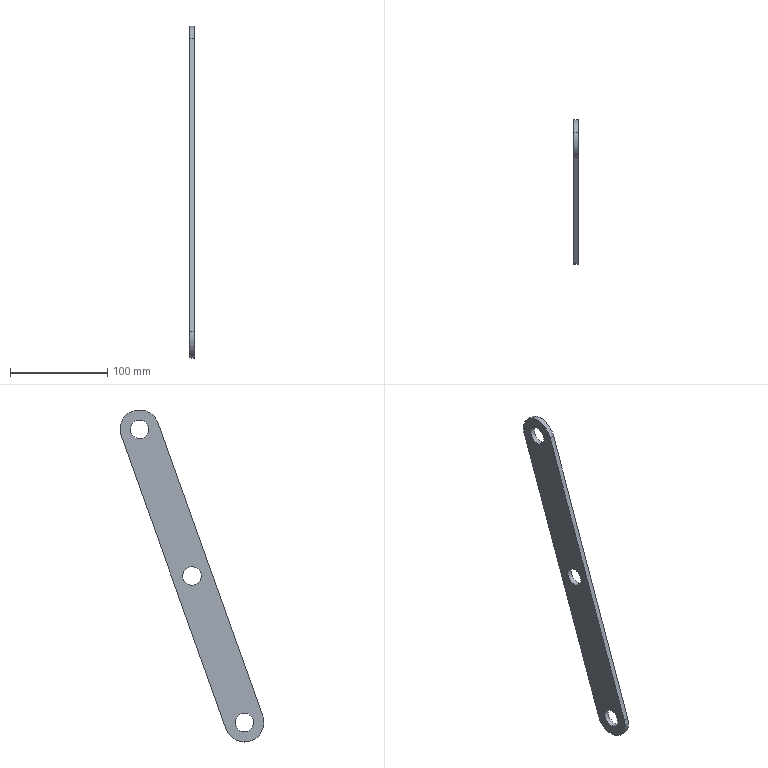Component | SolidWorks | ConnectingRod1-3 | 1 solid | 13 faces | box 5 x 147.82 x 341.29 mm | volume 66030 mm3 | cylinder 9 | plane 4 | commonest cylinder face diameters 19 x6 40 x3
STEP:
#1=CARTESIAN_POINT('',(-7.638,3.036,9.402));
#2=VERTEX_POINT('',#1);
#3=CARTESIAN_POINT('',(-7.638,2.784,8.697));
#4=VERTEX_POINT('',#3);
#5=CARTESIAN_POINT('',(-7.638,2.91,9.049));
#6=DIRECTION('',(1.,-0.,-0.));
#7=DIRECTION('',(0.,0.3369,0.9415));
#8=AXIS2_PLACEMENT_3D('',#5,#6,#7);
#9=CIRCLE('',#8,0.374);
#10=EDGE_CURVE('',#2,#4,#9,.T.);
#11=ORIENTED_EDGE('',*,*,#10,.T.);
#12=CARTESIAN_POINT('',(-7.835,2.784,8.697));
#13=VERTEX_POINT('',#12);
#14=CARTESIAN_POINT('',(-6.58,2.784,8.697));
#15=DIRECTION('',(-1.,0.,0.));
#16=VECTOR('',#15,39.37);
#17=LINE('',#14,#16);
#18=EDGE_CURVE('',#4,#13,#17,.T.);
#19=ORIENTED_EDGE('',*,*,#18,.T.);
#20=CARTESIAN_POINT('',(-7.835,3.036,9.402));
#21=VERTEX_POINT('',#20);
#22=CARTESIAN_POINT('',(-7.835,2.91,9.049));
#23=DIRECTION('',(-1.,0.,0.));
#24=DIRECTION('',(0.,0.3369,0.9415));
#25=AXIS2_PLACEMENT_3D('',#22,#23,#24);
#26=CIRCLE('',#25,0.374);
#27=EDGE_CURVE('',#13,#21,#26,.T.);
#28=ORIENTED_EDGE('',*,*,#27,.T.);
#29=CARTESIAN_POINT('',(-6.58,3.036,9.402));
#30=DIRECTION('',(-1.,0.,0.));
#31=VECTOR('',#30,39.37);
#32=LINE('',#29,#31);
#33=EDGE_CURVE('',#2,#21,#32,.T.);
#34=ORIENTED_EDGE('',*,*,#33,.F.);
#35=EDGE_LOOP('',(#11,#19,#28,#34));
#36=FACE_OUTER_BOUND('',#35,.T.);
#37=CARTESIAN_POINT('',(-6.58,2.91,9.049));
#38=DIRECTION('',(-1.,0.,0.));
#39=DIRECTION('',(0.,0.3369,0.9415));
#40=AXIS2_PLACEMENT_3D('',#37,#38,#39);
#41=CYLINDRICAL_SURFACE('',#40,0.374);
#42=ADVANCED_FACE('',(#36),#41,.F.);
#43=CARTESIAN_POINT('',(-7.638,0.9134,3.471));
#44=VERTEX_POINT('',#43);
#45=CARTESIAN_POINT('',(-7.638,0.6614,2.766));
#46=VERTEX_POINT('',#45);
#47=CARTESIAN_POINT('',(-7.638,0.7874,3.119));
#48=DIRECTION('',(1.,-0.,-0.));
#49=DIRECTION('',(0.,0.3369,0.9415));
#50=AXIS2_PLACEMENT_3D('',#47,#48,#49);
#51=CIRCLE('',#50,0.374);
#52=EDGE_CURVE('',#44,#46,#51,.T.);
#53=ORIENTED_EDGE('',*,*,#52,.T.);
#54=CARTESIAN_POINT('',(-7.835,0.6614,2.766));
#55=VERTEX_POINT('',#54);
#56=CARTESIAN_POINT('',(-6.58,0.6614,2.766));
#57=DIRECTION('',(-1.,0.,0.));
#58=VECTOR('',#57,39.37);
#59=LINE('',#56,#58);
#60=EDGE_CURVE('',#46,#55,#59,.T.);
#61=ORIENTED_EDGE('',*,*,#60,.T.);
#62=CARTESIAN_POINT('',(-7.835,0.9134,3.471));
#63=VERTEX_POINT('',#62);
#64=CARTESIAN_POINT('',(-7.835,0.7874,3.119));
#65=DIRECTION('',(-1.,0.,0.));
#66=DIRECTION('',(-0.,-0.3369,-0.9415));
#67=AXIS2_PLACEMENT_3D('',#64,#65,#66);
#68=CIRCLE('',#67,0.374);
#69=EDGE_CURVE('',#55,#63,#68,.T.);
#70=ORIENTED_EDGE('',*,*,#69,.T.);
#71=CARTESIAN_POINT('',(-6.58,0.9134,3.471));
#72=DIRECTION('',(-1.,0.,0.));
#73=VECTOR('',#72,39.37);
#74=LINE('',#71,#73);
#75=EDGE_CURVE('',#44,#63,#74,.T.);
#76=ORIENTED_EDGE('',*,*,#75,.F.);
#77=EDGE_LOOP('',(#53,#61,#70,#76));
#78=FACE_OUTER_BOUND('',#77,.T.);
#79=CARTESIAN_POINT('',(-6.58,0.7874,3.119));
#80=DIRECTION('',(-1.,0.,0.));
#81=DIRECTION('',(0.,0.3369,0.9415));
#82=AXIS2_PLACEMENT_3D('',#79,#80,#81);
#83=CYLINDRICAL_SURFACE('',#82,0.374);
#84=ADVANCED_FACE('',(#78),#83,.F.);
#85=CARTESIAN_POINT('',(-7.638,5.158,15.332));
#86=VERTEX_POINT('',#85);
#87=CARTESIAN_POINT('',(-7.638,4.906,14.628));
#88=VERTEX_POINT('',#87);
#89=CARTESIAN_POINT('',(-7.638,5.032,14.98));
#90=DIRECTION('',(1.,-0.,-0.));
#91=DIRECTION('',(0.,0.3369,0.9415));
#92=AXIS2_PLACEMENT_3D('',#89,#90,#91);
#93=CIRCLE('',#92,0.374);
#94=EDGE_CURVE('',#86,#88,#93,.T.);
#95=ORIENTED_EDGE('',*,*,#94,.T.);
#96=CARTESIAN_POINT('',(-7.835,4.906,14.628));
#97=VERTEX_POINT('',#96);
#98=CARTESIAN_POINT('',(-6.58,4.906,14.628));
#99=DIRECTION('',(-1.,0.,0.));
#100=VECTOR('',#99,39.37);
#101=LINE('',#98,#100);
#102=EDGE_CURVE('',#88,#97,#101,.T.);
#103=ORIENTED_EDGE('',*,*,#102,.T.);
#104=CARTESIAN_POINT('',(-7.835,5.158,15.332));
#105=VERTEX_POINT('',#104);
#106=CARTESIAN_POINT('',(-7.835,5.032,14.98));
#107=DIRECTION('',(-1.,0.,0.));
#108=DIRECTION('',(0.,0.3369,0.9415));
#109=AXIS2_PLACEMENT_3D('',#106,#107,#108);
#110=CIRCLE('',#109,0.374);
#111=EDGE_CURVE('',#97,#105,#110,.T.);
#112=ORIENTED_EDGE('',*,*,#111,.T.);
#113=CARTESIAN_POINT('',(-6.58,5.158,15.332));
#114=DIRECTION('',(-1.,0.,0.));
#115=VECTOR('',#114,39.37);
#116=LINE('',#113,#115);
#117=EDGE_CURVE('',#86,#105,#116,.T.);
#118=ORIENTED_EDGE('',*,*,#117,.F.);
#119=EDGE_LOOP('',(#95,#103,#112,#118));
#120=FACE_OUTER_BOUND('',#119,.T.);
#121=CARTESIAN_POINT('',(-6.58,5.032,14.98));
#122=DIRECTION('',(-1.,0.,0.));
#123=DIRECTION('',(0.,0.3369,0.9415));
#124=AXIS2_PLACEMENT_3D('',#121,#122,#123);
#125=CYLINDRICAL_SURFACE('',#124,0.374);
#126=ADVANCED_FACE('',(#120),#125,.F.);
#127=CARTESIAN_POINT('',(-7.638,4.291,15.246));
#128=VERTEX_POINT('',#127);
#129=CARTESIAN_POINT('',(-7.638,5.298,15.722));
#130=VERTEX_POINT('',#129);
#131=CARTESIAN_POINT('',(-7.638,5.032,14.98));
#132=DIRECTION('',(-1.,0.,0.));
#133=DIRECTION('',(0.,0.3369,0.9415));
#134=AXIS2_PLACEMENT_3D('',#131,#132,#133);
#135=CIRCLE('',#134,0.7874);
#136=EDGE_CURVE('',#128,#130,#135,.T.);
#137=ORIENTED_EDGE('',*,*,#136,.T.);
#138=CARTESIAN_POINT('',(-7.835,5.298,15.722));
#139=VERTEX_POINT('',#138);
#140=CARTESIAN_POINT('',(-7.638,5.298,15.722));
#141=DIRECTION('',(-1.,0.,0.));
#142=VECTOR('',#141,39.37);
#143=LINE('',#140,#142);
#144=EDGE_CURVE('',#130,#139,#143,.T.);
#145=ORIENTED_EDGE('',*,*,#144,.T.);
#146=CARTESIAN_POINT('',(-7.835,4.291,15.246));
#147=VERTEX_POINT('',#146);
#148=CARTESIAN_POINT('',(-7.835,5.032,14.98));
#149=DIRECTION('',(-1.,0.,0.));
#150=DIRECTION('',(0.,0.3369,0.9415));
#151=AXIS2_PLACEMENT_3D('',#148,#149,#150);
#152=CIRCLE('',#151,0.7874);
#153=EDGE_CURVE('',#147,#139,#152,.T.);
#154=ORIENTED_EDGE('',*,*,#153,.F.);
#155=CARTESIAN_POINT('',(-7.638,4.291,15.246));
#156=DIRECTION('',(-1.,0.,0.));
#157=VECTOR('',#156,39.37);
#158=LINE('',#155,#157);
#159=EDGE_CURVE('',#128,#147,#158,.T.);
#160=ORIENTED_EDGE('',*,*,#159,.F.);
#161=EDGE_LOOP('',(#137,#145,#154,#160));
#162=FACE_OUTER_BOUND('',#161,.T.);
#163=CARTESIAN_POINT('',(-7.638,5.032,14.98));
#164=DIRECTION('',(-1.,0.,0.));
#165=DIRECTION('',(0.,0.3369,0.9415));
#166=AXIS2_PLACEMENT_3D('',#163,#164,#165);
#167=CYLINDRICAL_SURFACE('',#166,0.7874);
#168=ADVANCED_FACE('',(#162),#167,.T.);
#169=CARTESIAN_POINT('',(-7.835,1.529,2.853));
#170=VERTEX_POINT('',#169);
#171=CARTESIAN_POINT('',(-7.835,0.04604,3.384));
#172=VERTEX_POINT('',#171);
#173=CARTESIAN_POINT('',(-7.835,0.7874,3.119));
#174=DIRECTION('',(-1.,0.,0.));
#175=DIRECTION('',(0.,0.3369,0.9415));
#176=AXIS2_PLACEMENT_3D('',#173,#174,#175);
#177=CIRCLE('',#176,0.7874);
#178=EDGE_CURVE('',#170,#172,#177,.T.);
#179=ORIENTED_EDGE('',*,*,#178,.F.);
#180=CARTESIAN_POINT('',(-7.638,1.529,2.853));
#181=VERTEX_POINT('',#180);
#182=CARTESIAN_POINT('',(-7.638,1.529,2.853));
#183=DIRECTION('',(-1.,0.,0.));
#184=VECTOR('',#183,39.37);
#185=LINE('',#182,#184);
#186=EDGE_CURVE('',#181,#170,#185,.T.);
#187=ORIENTED_EDGE('',*,*,#186,.F.);
#188=CARTESIAN_POINT('',(-7.638,0.04604,3.384));
#189=VERTEX_POINT('',#188);
#190=CARTESIAN_POINT('',(-7.638,0.7874,3.119));
#191=DIRECTION('',(-1.,0.,0.));
#192=DIRECTION('',(0.,0.3369,0.9415));
#193=AXIS2_PLACEMENT_3D('',#190,#191,#192);
#194=CIRCLE('',#193,0.7874);
#195=EDGE_CURVE('',#181,#189,#194,.T.);
#196=ORIENTED_EDGE('',*,*,#195,.T.);
#197=CARTESIAN_POINT('',(-7.638,0.04604,3.384));
#198=DIRECTION('',(-1.,0.,0.));
#199=VECTOR('',#198,39.37);
#200=LINE('',#197,#199);
#201=EDGE_CURVE('',#189,#172,#200,.T.);
#202=ORIENTED_EDGE('',*,*,#201,.T.);
#203=EDGE_LOOP('',(#179,#187,#196,#202));
#204=FACE_OUTER_BOUND('',#203,.T.);
#205=CARTESIAN_POINT('',(-7.638,0.7874,3.119));
#206=DIRECTION('',(-1.,0.,0.));
#207=DIRECTION('',(0.,0.3369,0.9415));
#208=AXIS2_PLACEMENT_3D('',#205,#206,#207);
#209=CYLINDRICAL_SURFACE('',#208,0.7874);
#210=ADVANCED_FACE('',(#204),#209,.T.);
#211=CARTESIAN_POINT('',(-7.835,5.774,14.715));
#212=VERTEX_POINT('',#211);
#213=CARTESIAN_POINT('',(-7.835,1.529,2.853));
#214=DIRECTION('',(-0.,-0.3369,-0.9415));
#215=VECTOR('',#214,39.37);
#216=LINE('',#213,#215);
#217=EDGE_CURVE('',#212,#170,#216,.T.);
#218=ORIENTED_EDGE('',*,*,#217,.F.);
#219=CARTESIAN_POINT('',(-7.638,5.774,14.715));
#220=VERTEX_POINT('',#219);
#221=CARTESIAN_POINT('',(-7.638,5.774,14.715));
#222=DIRECTION('',(-1.,0.,0.));
#223=VECTOR('',#222,39.37);
#224=LINE('',#221,#223);
#225=EDGE_CURVE('',#220,#212,#224,.T.);
#226=ORIENTED_EDGE('',*,*,#225,.F.);
#227=CARTESIAN_POINT('',(-7.638,1.529,2.853));
#228=DIRECTION('',(-0.,-0.3369,-0.9415));
#229=VECTOR('',#228,39.37);
#230=LINE('',#227,#229);
#231=EDGE_CURVE('',#220,#181,#230,.T.);
#232=ORIENTED_EDGE('',*,*,#231,.T.);
#233=ORIENTED_EDGE('',*,*,#186,.T.);
#234=EDGE_LOOP('',(#218,#226,#232,#233));
#235=FACE_OUTER_BOUND('',#234,.T.);
#236=CARTESIAN_POINT('',(-7.638,1.529,2.853));
#237=DIRECTION('',(-0.,0.9415,-0.3369));
#238=DIRECTION('',(-0.,-0.3369,-0.9415));
#239=AXIS2_PLACEMENT_3D('',#236,#237,#238);
#240=PLANE('',#239);
#241=ADVANCED_FACE('',(#235),#240,.T.);
#242=ORIENTED_EDGE('',*,*,#144,.F.);
#243=CARTESIAN_POINT('',(-7.638,5.032,14.98));
#244=DIRECTION('',(-1.,0.,0.));
#245=DIRECTION('',(0.,0.3369,0.9415));
#246=AXIS2_PLACEMENT_3D('',#243,#244,#245);
#247=CIRCLE('',#246,0.7874);
#248=EDGE_CURVE('',#130,#220,#247,.T.);
#249=ORIENTED_EDGE('',*,*,#248,.T.);
#250=ORIENTED_EDGE('',*,*,#225,.T.);
#251=CARTESIAN_POINT('',(-7.835,5.032,14.98));
#252=DIRECTION('',(-1.,0.,0.));
#253=DIRECTION('',(0.,0.3369,0.9415));
#254=AXIS2_PLACEMENT_3D('',#251,#252,#253);
#255=CIRCLE('',#254,0.7874);
#256=EDGE_CURVE('',#139,#212,#255,.T.);
#257=ORIENTED_EDGE('',*,*,#256,.F.);
#258=EDGE_LOOP('',(#242,#249,#250,#257));
#259=FACE_OUTER_BOUND('',#258,.T.);
#260=CARTESIAN_POINT('',(-7.638,5.032,14.98));
#261=DIRECTION('',(-1.,0.,0.));
#262=DIRECTION('',(0.,0.3369,0.9415));
#263=AXIS2_PLACEMENT_3D('',#260,#261,#262);
#264=CYLINDRICAL_SURFACE('',#263,0.7874);
#265=ADVANCED_FACE('',(#259),#264,.T.);
#266=CARTESIAN_POINT('',(-7.835,0.04604,3.384));
#267=DIRECTION('',(0.,0.3369,0.9415));
#268=VECTOR('',#267,39.37);
#269=LINE('',#266,#268);
#270=EDGE_CURVE('',#172,#147,#269,.T.);
#271=ORIENTED_EDGE('',*,*,#270,.F.);
#272=ORIENTED_EDGE('',*,*,#201,.F.);
#273=CARTESIAN_POINT('',(-7.638,0.04604,3.384));
#274=DIRECTION('',(0.,0.3369,0.9415));
#275=VECTOR('',#274,39.37);
#276=LINE('',#273,#275);
#277=EDGE_CURVE('',#189,#128,#276,.T.);
#278=ORIENTED_EDGE('',*,*,#277,.T.);
#279=ORIENTED_EDGE('',*,*,#159,.T.);
#280=EDGE_LOOP('',(#271,#272,#278,#279));
#281=FACE_OUTER_BOUND('',#280,.T.);
#282=CARTESIAN_POINT('',(-7.638,0.04604,3.384));
#283=DIRECTION('',(0.,-0.9415,0.3369));
#284=DIRECTION('',(0.,0.3369,0.9415));
#285=AXIS2_PLACEMENT_3D('',#282,#283,#284);
#286=PLANE('',#285);
#287=ADVANCED_FACE('',(#281),#286,.T.);
#288=ORIENTED_EDGE('',*,*,#10,.F.);
#289=CARTESIAN_POINT('',(-7.638,2.91,9.049));
#290=DIRECTION('',(1.,-0.,-0.));
#291=DIRECTION('',(0.,0.3369,0.9415));
#292=AXIS2_PLACEMENT_3D('',#289,#290,#291);
#293=CIRCLE('',#292,0.374);
#294=EDGE_CURVE('',#4,#2,#293,.T.);
#295=ORIENTED_EDGE('',*,*,#294,.F.);
#296=EDGE_LOOP('',(#288,#295));
#297=FACE_BOUND('',#296,.T.);
#298=ORIENTED_EDGE('',*,*,#52,.F.);
#299=CARTESIAN_POINT('',(-7.638,0.7874,3.119));
#300=DIRECTION('',(1.,-0.,-0.));
#301=DIRECTION('',(0.,0.3369,0.9415));
#302=AXIS2_PLACEMENT_3D('',#299,#300,#301);
#303=CIRCLE('',#302,0.374);
#304=EDGE_CURVE('',#46,#44,#303,.T.);
#305=ORIENTED_EDGE('',*,*,#304,.F.);
#306=EDGE_LOOP('',(#298,#305));
#307=FACE_BOUND('',#306,.T.);
#308=ORIENTED_EDGE('',*,*,#94,.F.);
#309=CARTESIAN_POINT('',(-7.638,5.032,14.98));
#310=DIRECTION('',(1.,-0.,-0.));
#311=DIRECTION('',(0.,0.3369,0.9415));
#312=AXIS2_PLACEMENT_3D('',#309,#310,#311);
#313=CIRCLE('',#312,0.374);
#314=EDGE_CURVE('',#88,#86,#313,.T.);
#315=ORIENTED_EDGE('',*,*,#314,.F.);
#316=EDGE_LOOP('',(#308,#315));
#317=FACE_BOUND('',#316,.T.);
#318=ORIENTED_EDGE('',*,*,#195,.F.);
#319=ORIENTED_EDGE('',*,*,#231,.F.);
#320=ORIENTED_EDGE('',*,*,#248,.F.);
#321=ORIENTED_EDGE('',*,*,#136,.F.);
#322=ORIENTED_EDGE('',*,*,#277,.F.);
#323=EDGE_LOOP('',(#318,#319,#320,#321,#322));
#324=FACE_OUTER_BOUND('',#323,.T.);
#325=CARTESIAN_POINT('',(-7.638,0.7874,3.119));
#326=DIRECTION('',(-1.,0.,0.));
#327=DIRECTION('',(0.,0.3369,0.9415));
#328=AXIS2_PLACEMENT_3D('',#325,#326,#327);
#329=PLANE('',#328);
#330=ADVANCED_FACE('',(#297,#307,#317,#324),#329,.F.);
#331=CARTESIAN_POINT('',(-7.835,2.91,9.049));
#332=DIRECTION('',(-1.,0.,0.));
#333=DIRECTION('',(0.,0.3369,0.9415));
#334=AXIS2_PLACEMENT_3D('',#331,#332,#333);
#335=CIRCLE('',#334,0.374);
#336=EDGE_CURVE('',#21,#13,#335,.T.);
#337=ORIENTED_EDGE('',*,*,#336,.F.);
#338=ORIENTED_EDGE('',*,*,#27,.F.);
#339=EDGE_LOOP('',(#337,#338));
#340=FACE_BOUND('',#339,.T.);
#341=CARTESIAN_POINT('',(-7.835,0.7874,3.119));
#342=DIRECTION('',(-1.,0.,0.));
#343=DIRECTION('',(-0.,-0.3369,-0.9415));
#344=AXIS2_PLACEMENT_3D('',#341,#342,#343);
#345=CIRCLE('',#344,0.374);
#346=EDGE_CURVE('',#63,#55,#345,.T.);
#347=ORIENTED_EDGE('',*,*,#346,.F.);
#348=ORIENTED_EDGE('',*,*,#69,.F.);
#349=EDGE_LOOP('',(#347,#348));
#350=FACE_BOUND('',#349,.T.);
#351=CARTESIAN_POINT('',(-7.835,5.032,14.98));
#352=DIRECTION('',(-1.,0.,0.));
#353=DIRECTION('',(0.,0.3369,0.9415));
#354=AXIS2_PLACEMENT_3D('',#351,#352,#353);
#355=CIRCLE('',#354,0.374);
#356=EDGE_CURVE('',#105,#97,#355,.T.);
#357=ORIENTED_EDGE('',*,*,#356,.F.);
#358=ORIENTED_EDGE('',*,*,#111,.F.);
#359=EDGE_LOOP('',(#357,#358));
#360=FACE_BOUND('',#359,.T.);
#361=ORIENTED_EDGE('',*,*,#178,.T.);
#362=ORIENTED_EDGE('',*,*,#270,.T.);
#363=ORIENTED_EDGE('',*,*,#153,.T.);
#364=ORIENTED_EDGE('',*,*,#256,.T.);
#365=ORIENTED_EDGE('',*,*,#217,.T.);
#366=EDGE_LOOP('',(#361,#362,#363,#364,#365));
#367=FACE_OUTER_BOUND('',#366,.T.);
#368=CARTESIAN_POINT('',(-7.835,0.7874,3.119));
#369=DIRECTION('',(-1.,0.,0.));
#370=DIRECTION('',(0.,0.3369,0.9415));
#371=AXIS2_PLACEMENT_3D('',#368,#369,#370);
#372=PLANE('',#371);
#373=ADVANCED_FACE('',(#340,#350,#360,#367),#372,.T.);
#374=ORIENTED_EDGE('',*,*,#102,.F.);
#375=ORIENTED_EDGE('',*,*,#314,.T.);
#376=ORIENTED_EDGE('',*,*,#117,.T.);
#377=ORIENTED_EDGE('',*,*,#356,.T.);
#378=EDGE_LOOP('',(#374,#375,#376,#377));
#379=FACE_OUTER_BOUND('',#378,.T.);
#380=CARTESIAN_POINT('',(-6.58,5.032,14.98));
#381=DIRECTION('',(-1.,0.,0.));
#382=DIRECTION('',(0.,0.3369,0.9415));
#383=AXIS2_PLACEMENT_3D('',#380,#381,#382);
#384=CYLINDRICAL_SURFACE('',#383,0.374);
#385=ADVANCED_FACE('',(#379),#384,.F.);
#386=ORIENTED_EDGE('',*,*,#60,.F.);
#387=ORIENTED_EDGE('',*,*,#304,.T.);
#388=ORIENTED_EDGE('',*,*,#75,.T.);
#389=ORIENTED_EDGE('',*,*,#346,.T.);
#390=EDGE_LOOP('',(#386,#387,#388,#389));
#391=FACE_OUTER_BOUND('',#390,.T.);
#392=CARTESIAN_POINT('',(-6.58,0.7874,3.119));
#393=DIRECTION('',(-1.,0.,0.));
#394=DIRECTION('',(0.,0.3369,0.9415));
#395=AXIS2_PLACEMENT_3D('',#392,#393,#394);
#396=CYLINDRICAL_SURFACE('',#395,0.374);
#397=ADVANCED_FACE('',(#391),#396,.F.);
#398=ORIENTED_EDGE('',*,*,#18,.F.);
#399=ORIENTED_EDGE('',*,*,#294,.T.);
#400=ORIENTED_EDGE('',*,*,#33,.T.);
#401=ORIENTED_EDGE('',*,*,#336,.T.);
#402=EDGE_LOOP('',(#398,#399,#400,#401));
#403=FACE_OUTER_BOUND('',#402,.T.);
#404=CARTESIAN_POINT('',(-6.58,2.91,9.049));
#405=DIRECTION('',(-1.,0.,0.));
#406=DIRECTION('',(0.,0.3369,0.9415));
#407=AXIS2_PLACEMENT_3D('',#404,#405,#406);
#408=CYLINDRICAL_SURFACE('',#407,0.374);
#409=ADVANCED_FACE('',(#403),#408,.F.);
#410=CLOSED_SHELL('',(#42,#84,#126,#168,#210,#241,#265,#287,#330,#373,#385,#397,#409));
#411=MANIFOLD_SOLID_BREP('',#410);
#412=CARTESIAN_POINT('',(0.,0.,0.));
#413=DIRECTION('',(0.,0.,1.));
#414=DIRECTION('',(1.,0.,0.));
#415=AXIS2_PLACEMENT_3D('',#412,#413,#414);
#416=(LENGTH_UNIT()NAMED_UNIT(*)SI_UNIT($,.METRE.));
#417=LENGTH_MEASURE_WITH_UNIT(LENGTH_MEASURE(0.0254),#416);
#418=DIMENSIONAL_EXPONENTS(1.,0.,0.,0.,0.,0.,0.);
#419=(CONVERSION_BASED_UNIT('',#417)LENGTH_UNIT()NAMED_UNIT(#418));
#420=UNCERTAINTY_MEASURE_WITH_UNIT(LENGTH_MEASURE(0.00001),#419,'','');
#421=(NAMED_UNIT(*)PLANE_ANGLE_UNIT()SI_UNIT($,.RADIAN.));
#422=(NAMED_UNIT(*)SI_UNIT($,.STERADIAN.)SOLID_ANGLE_UNIT());
#423=(GEOMETRIC_REPRESENTATION_CONTEXT(3)GLOBAL_UNCERTAINTY_ASSIGNED_CONTEXT((#420))GLOBAL_UNIT_ASSIGNED_CONTEXT((#419,#421,#422))REPRESENTATION_CONTEXT('',''));
#424=ADVANCED_BREP_SHAPE_REPRESENTATION('',(#411,#415),#423);
#425=COLOUR_RGB('',0.7922,0.8196,0.9333);
#426=FILL_AREA_STYLE_COLOUR('',#425);
#427=FILL_AREA_STYLE('',(#426));
#428=SURFACE_STYLE_FILL_AREA(#427);
#429=SURFACE_SIDE_STYLE('',(#428));
#430=SURFACE_STYLE_USAGE(.BOTH.,#429);
#431=PRESENTATION_STYLE_ASSIGNMENT((#430));
#432=STYLED_ITEM('',(#431),#411);
#433=(LENGTH_UNIT()NAMED_UNIT(*)SI_UNIT($,.METRE.));
#434=LENGTH_MEASURE_WITH_UNIT(LENGTH_MEASURE(0.0254),#433);
#435=DIMENSIONAL_EXPONENTS(1.,0.,0.,0.,0.,0.,0.);
#436=(CONVERSION_BASED_UNIT('',#434)LENGTH_UNIT()NAMED_UNIT(#435));
#437=UNCERTAINTY_MEASURE_WITH_UNIT(LENGTH_MEASURE(0.00001),#436,'','');
#438=(NAMED_UNIT(*)PLANE_ANGLE_UNIT()SI_UNIT($,.RADIAN.));
#439=(NAMED_UNIT(*)SI_UNIT($,.STERADIAN.)SOLID_ANGLE_UNIT());
#440=(GEOMETRIC_REPRESENTATION_CONTEXT(3)GLOBAL_UNCERTAINTY_ASSIGNED_CONTEXT((#437))GLOBAL_UNIT_ASSIGNED_CONTEXT((#436,#438,#439))REPRESENTATION_CONTEXT('',''));
#441=MECHANICAL_DESIGN_GEOMETRIC_PRESENTATION_REPRESENTATION('',(#432),#440);
#442=PRESENTATION_LAYER_ASSIGNMENT('','',(#432));